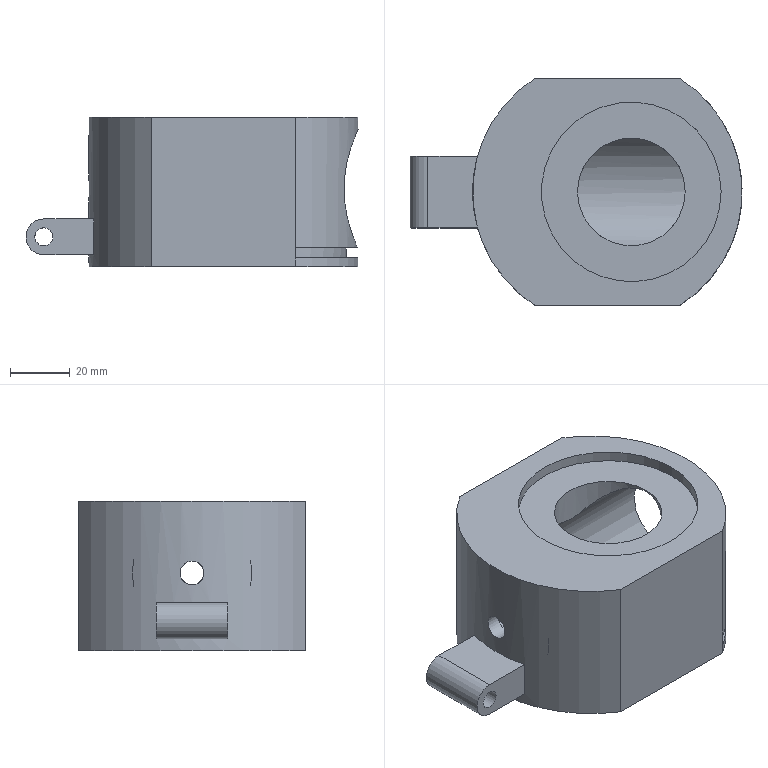Component | NX | SHEJI_-2 | 1 solid | 28 faces | volume 181165 mm3 | plane 18 | cylinder 10 | commonest cylinder face diameters 90 x3 40 x1 36 x1 12 x1 6 x1 8 x1 60 x1 82 x1